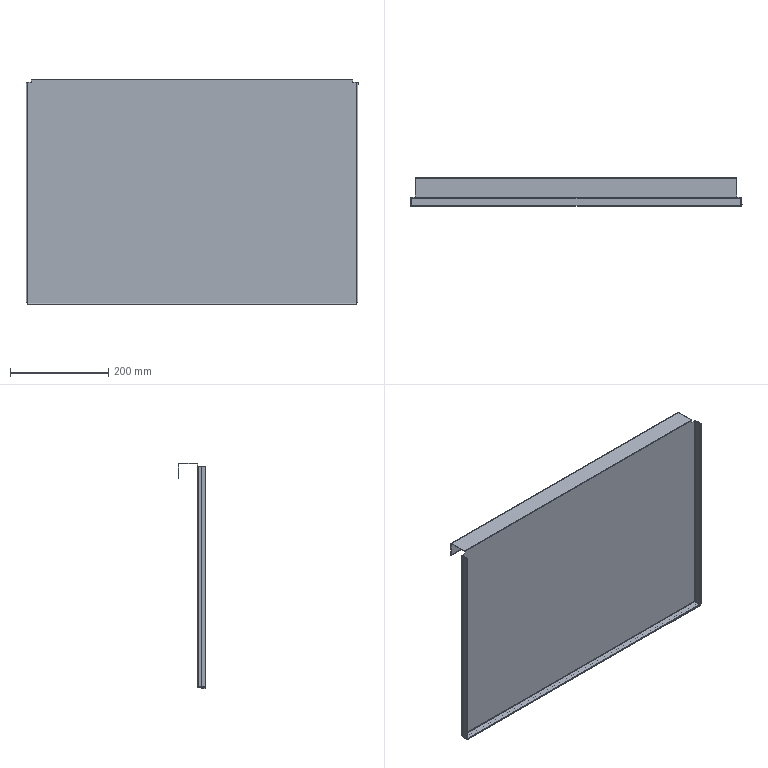Component | SolidWorks | PC-CAJ-P08-1_PM-CAJ-P33-1 | 1 solid | 78 faces | volume 272826 mm3 | plane 62 | cylinder 16 | commonest cylinder face diameters 1 x5 2.4 x5 2.7 x3 1.3 x3 | material Plain Carbon Steel